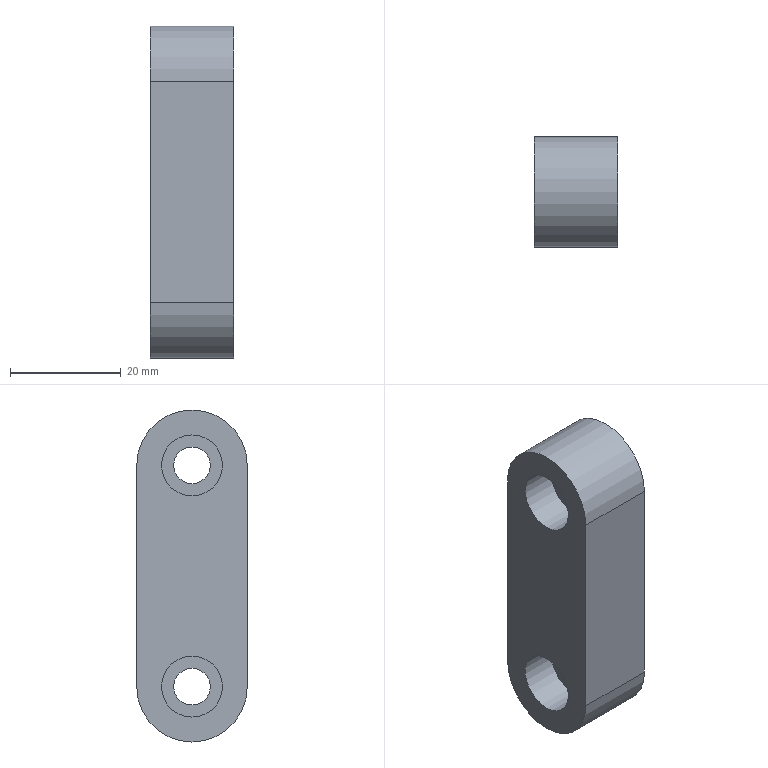Component | NX | SLIDER | 1 solid | 12 faces | box 15 x 20 x 60 mm | volume 14859 mm3 | plane 6 | cylinder 6 | commonest cylinder face diameters 6.6 x2 11 x2 20 x2
STEP:
#1=CARTESIAN_POINT('',(0.,0.,0.));
#2=DIRECTION('',(0.,0.,1.));
#3=DIRECTION('',(1.,0.,0.));
#4=AXIS2_PLACEMENT_3D('',#1,#2,#3);
#5=CARTESIAN_POINT('',(495.625,-9.909,-94.557));
#6=VERTEX_POINT('',#5);
#7=CARTESIAN_POINT('',(495.625,-9.909,-134.557));
#8=VERTEX_POINT('',#7);
#9=CARTESIAN_POINT('',(495.625,-9.909,-84.557));
#10=DIRECTION('',(0.,0.,-1.));
#11=VECTOR('',#10,1.);
#12=LINE('',#9,#11);
#13=CARTESIAN_POINT('',(510.625,-9.909,-84.557));
#14=DIRECTION('',(0.,1.,0.));
#15=DIRECTION('',(0.,0.,1.));
#16=AXIS2_PLACEMENT_3D('',#13,#14,#15);
#17=PLANE('',#16);
#18=CARTESIAN_POINT('',(0.,-15.));
#19=DIRECTION('',(-1.,0.));
#20=VECTOR('',#19,1.);
#21=LINE('',#18,#20);
#22=(GEOMETRIC_REPRESENTATION_CONTEXT(2)PARAMETRIC_REPRESENTATION_CONTEXT()REPRESENTATION_CONTEXT('',''));
#23=DEFINITIONAL_REPRESENTATION('',(#21),#22);
#24=PCURVE('',#17,#23);
#25=CARTESIAN_POINT('',(495.625,0.09065,-114.557));
#26=DIRECTION('',(1.,0.,0.));
#27=DIRECTION('',(0.,0.,-1.));
#28=AXIS2_PLACEMENT_3D('',#25,#26,#27);
#29=PLANE('',#28);
#30=CARTESIAN_POINT('',(-30.,-10.));
#31=DIRECTION('',(1.,0.));
#32=VECTOR('',#31,1.);
#33=LINE('',#30,#32);
#34=(GEOMETRIC_REPRESENTATION_CONTEXT(2)PARAMETRIC_REPRESENTATION_CONTEXT()REPRESENTATION_CONTEXT('',''));
#35=DEFINITIONAL_REPRESENTATION('',(#33),#34);
#36=PCURVE('',#29,#35);
#37=SURFACE_CURVE('',#12,(#24,#36),.PCURVE_S1.);
#38=EDGE_CURVE('',#6,#8,#37,.T.);
#39=ORIENTED_EDGE('',*,*,#38,.T.);
#40=CARTESIAN_POINT('',(510.625,-9.909,-134.557));
#41=VERTEX_POINT('',#40);
#42=CARTESIAN_POINT('',(510.625,-9.909,-134.557));
#43=DIRECTION('',(1.,0.,0.));
#44=VECTOR('',#43,1.);
#45=LINE('',#42,#44);
#46=CARTESIAN_POINT('',(-50.,0.));
#47=DIRECTION('',(0.,1.));
#48=VECTOR('',#47,1.);
#49=LINE('',#46,#48);
#50=(GEOMETRIC_REPRESENTATION_CONTEXT(2)PARAMETRIC_REPRESENTATION_CONTEXT()REPRESENTATION_CONTEXT('',''));
#51=DEFINITIONAL_REPRESENTATION('',(#49),#50);
#52=PCURVE('',#17,#51);
#53=CARTESIAN_POINT('',(510.625,0.09065,-134.557));
#54=DIRECTION('',(-1.,0.,0.));
#55=DIRECTION('',(0.,0.,1.));
#56=AXIS2_PLACEMENT_3D('',#53,#54,#55);
#57=CYLINDRICAL_SURFACE('',#56,10.);
#58=CARTESIAN_POINT('',(4.712,0.));
#59=DIRECTION('',(0.,-1.));
#60=VECTOR('',#59,1.);
#61=LINE('',#58,#60);
#62=(GEOMETRIC_REPRESENTATION_CONTEXT(2)PARAMETRIC_REPRESENTATION_CONTEXT()REPRESENTATION_CONTEXT('',''));
#63=DEFINITIONAL_REPRESENTATION('',(#61),#62);
#64=PCURVE('',#57,#63);
#65=SURFACE_CURVE('',#45,(#52,#64),.PCURVE_S1.);
#66=EDGE_CURVE('',#8,#41,#65,.T.);
#67=ORIENTED_EDGE('',*,*,#66,.T.);
#68=CARTESIAN_POINT('',(510.625,-9.909,-94.557));
#69=VERTEX_POINT('',#68);
#70=CARTESIAN_POINT('',(510.625,-9.909,-84.557));
#71=DIRECTION('',(0.,0.,-1.));
#72=VECTOR('',#71,1.);
#73=LINE('',#70,#72);
#74=CARTESIAN_POINT('',(0.,0.));
#75=DIRECTION('',(-1.,0.));
#76=VECTOR('',#75,1.);
#77=LINE('',#74,#76);
#78=(GEOMETRIC_REPRESENTATION_CONTEXT(2)PARAMETRIC_REPRESENTATION_CONTEXT()REPRESENTATION_CONTEXT('',''));
#79=DEFINITIONAL_REPRESENTATION('',(#77),#78);
#80=PCURVE('',#17,#79);
#81=CARTESIAN_POINT('',(510.625,0.09065,-114.557));
#82=DIRECTION('',(1.,0.,0.));
#83=DIRECTION('',(0.,0.,-1.));
#84=AXIS2_PLACEMENT_3D('',#81,#82,#83);
#85=PLANE('',#84);
#86=CARTESIAN_POINT('',(-30.,-10.));
#87=DIRECTION('',(1.,0.));
#88=VECTOR('',#87,1.);
#89=LINE('',#86,#88);
#90=(GEOMETRIC_REPRESENTATION_CONTEXT(2)PARAMETRIC_REPRESENTATION_CONTEXT()REPRESENTATION_CONTEXT('',''));
#91=DEFINITIONAL_REPRESENTATION('',(#89),#90);
#92=PCURVE('',#85,#91);
#93=SURFACE_CURVE('',#73,(#80,#92),.PCURVE_S1.);
#94=EDGE_CURVE('',#69,#41,#93,.T.);
#95=ORIENTED_EDGE('',*,*,#94,.F.);
#96=CARTESIAN_POINT('',(510.625,-9.909,-94.557));
#97=DIRECTION('',(-1.,0.,0.));
#98=VECTOR('',#97,1.);
#99=LINE('',#96,#98);
#100=CARTESIAN_POINT('',(-10.,0.));
#101=DIRECTION('',(0.,-1.));
#102=VECTOR('',#101,1.);
#103=LINE('',#100,#102);
#104=(GEOMETRIC_REPRESENTATION_CONTEXT(2)PARAMETRIC_REPRESENTATION_CONTEXT()REPRESENTATION_CONTEXT('',''));
#105=DEFINITIONAL_REPRESENTATION('',(#103),#104);
#106=PCURVE('',#17,#105);
#107=CARTESIAN_POINT('',(510.625,0.09065,-94.557));
#108=DIRECTION('',(-1.,0.,0.));
#109=DIRECTION('',(0.,0.,1.));
#110=AXIS2_PLACEMENT_3D('',#107,#108,#109);
#111=CYLINDRICAL_SURFACE('',#110,10.);
#112=CARTESIAN_POINT('',(4.712,0.));
#113=DIRECTION('',(0.,1.));
#114=VECTOR('',#113,1.);
#115=LINE('',#112,#114);
#116=(GEOMETRIC_REPRESENTATION_CONTEXT(2)PARAMETRIC_REPRESENTATION_CONTEXT()REPRESENTATION_CONTEXT('',''));
#117=DEFINITIONAL_REPRESENTATION('',(#115),#116);
#118=PCURVE('',#111,#117);
#119=SURFACE_CURVE('',#99,(#106,#118),.PCURVE_S1.);
#120=EDGE_CURVE('',#69,#6,#119,.T.);
#121=ORIENTED_EDGE('',*,*,#120,.T.);
#122=EDGE_LOOP('',(#39,#67,#95,#121));
#123=FACE_BOUND('',#122,.T.);
#124=ADVANCED_FACE('',(#123),#17,.F.);
#125=CARTESIAN_POINT('',(510.625,10.091,-134.557));
#126=VERTEX_POINT('',#125);
#127=CARTESIAN_POINT('',(510.625,10.091,-94.557));
#128=VERTEX_POINT('',#127);
#129=CARTESIAN_POINT('',(510.625,10.091,-144.557));
#130=DIRECTION('',(0.,0.,1.));
#131=VECTOR('',#130,1.);
#132=LINE('',#129,#131);
#133=CARTESIAN_POINT('',(510.625,10.091,-144.557));
#134=DIRECTION('',(0.,-1.,0.));
#135=DIRECTION('',(0.,0.,-1.));
#136=AXIS2_PLACEMENT_3D('',#133,#134,#135);
#137=PLANE('',#136);
#138=CARTESIAN_POINT('',(0.,0.));
#139=DIRECTION('',(-1.,0.));
#140=VECTOR('',#139,1.);
#141=LINE('',#138,#140);
#142=(GEOMETRIC_REPRESENTATION_CONTEXT(2)PARAMETRIC_REPRESENTATION_CONTEXT()REPRESENTATION_CONTEXT('',''));
#143=DEFINITIONAL_REPRESENTATION('',(#141),#142);
#144=PCURVE('',#137,#143);
#145=CARTESIAN_POINT('',(30.,10.));
#146=DIRECTION('',(-1.,0.));
#147=VECTOR('',#146,1.);
#148=LINE('',#145,#147);
#149=(GEOMETRIC_REPRESENTATION_CONTEXT(2)PARAMETRIC_REPRESENTATION_CONTEXT()REPRESENTATION_CONTEXT('',''));
#150=DEFINITIONAL_REPRESENTATION('',(#148),#149);
#151=PCURVE('',#85,#150);
#152=SURFACE_CURVE('',#132,(#144,#151),.PCURVE_S1.);
#153=EDGE_CURVE('',#126,#128,#152,.T.);
#154=ORIENTED_EDGE('',*,*,#153,.F.);
#155=CARTESIAN_POINT('',(495.625,10.091,-134.557));
#156=VERTEX_POINT('',#155);
#157=CARTESIAN_POINT('',(510.625,10.091,-134.557));
#158=DIRECTION('',(-1.,0.,0.));
#159=VECTOR('',#158,1.);
#160=LINE('',#157,#159);
#161=CARTESIAN_POINT('',(-10.,0.));
#162=DIRECTION('',(0.,-1.));
#163=VECTOR('',#162,1.);
#164=LINE('',#161,#163);
#165=(GEOMETRIC_REPRESENTATION_CONTEXT(2)PARAMETRIC_REPRESENTATION_CONTEXT()REPRESENTATION_CONTEXT('',''));
#166=DEFINITIONAL_REPRESENTATION('',(#164),#165);
#167=PCURVE('',#137,#166);
#168=CARTESIAN_POINT('',(1.571,0.));
#169=DIRECTION('',(0.,1.));
#170=VECTOR('',#169,1.);
#171=LINE('',#168,#170);
#172=(GEOMETRIC_REPRESENTATION_CONTEXT(2)PARAMETRIC_REPRESENTATION_CONTEXT()REPRESENTATION_CONTEXT('',''));
#173=DEFINITIONAL_REPRESENTATION('',(#171),#172);
#174=PCURVE('',#57,#173);
#175=SURFACE_CURVE('',#160,(#167,#174),.PCURVE_S1.);
#176=EDGE_CURVE('',#126,#156,#175,.T.);
#177=ORIENTED_EDGE('',*,*,#176,.T.);
#178=CARTESIAN_POINT('',(495.625,10.091,-94.557));
#179=VERTEX_POINT('',#178);
#180=CARTESIAN_POINT('',(495.625,10.091,-144.557));
#181=DIRECTION('',(0.,0.,1.));
#182=VECTOR('',#181,1.);
#183=LINE('',#180,#182);
#184=CARTESIAN_POINT('',(0.,-15.));
#185=DIRECTION('',(-1.,0.));
#186=VECTOR('',#185,1.);
#187=LINE('',#184,#186);
#188=(GEOMETRIC_REPRESENTATION_CONTEXT(2)PARAMETRIC_REPRESENTATION_CONTEXT()REPRESENTATION_CONTEXT('',''));
#189=DEFINITIONAL_REPRESENTATION('',(#187),#188);
#190=PCURVE('',#137,#189);
#191=CARTESIAN_POINT('',(30.,10.));
#192=DIRECTION('',(-1.,0.));
#193=VECTOR('',#192,1.);
#194=LINE('',#191,#193);
#195=(GEOMETRIC_REPRESENTATION_CONTEXT(2)PARAMETRIC_REPRESENTATION_CONTEXT()REPRESENTATION_CONTEXT('',''));
#196=DEFINITIONAL_REPRESENTATION('',(#194),#195);
#197=PCURVE('',#29,#196);
#198=SURFACE_CURVE('',#183,(#190,#197),.PCURVE_S1.);
#199=EDGE_CURVE('',#156,#179,#198,.T.);
#200=ORIENTED_EDGE('',*,*,#199,.T.);
#201=CARTESIAN_POINT('',(510.625,10.091,-94.557));
#202=DIRECTION('',(1.,0.,0.));
#203=VECTOR('',#202,1.);
#204=LINE('',#201,#203);
#205=CARTESIAN_POINT('',(-50.,0.));
#206=DIRECTION('',(0.,1.));
#207=VECTOR('',#206,1.);
#208=LINE('',#205,#207);
#209=(GEOMETRIC_REPRESENTATION_CONTEXT(2)PARAMETRIC_REPRESENTATION_CONTEXT()REPRESENTATION_CONTEXT('',''));
#210=DEFINITIONAL_REPRESENTATION('',(#208),#209);
#211=PCURVE('',#137,#210);
#212=CARTESIAN_POINT('',(7.854,0.));
#213=DIRECTION('',(0.,-1.));
#214=VECTOR('',#213,1.);
#215=LINE('',#212,#214);
#216=(GEOMETRIC_REPRESENTATION_CONTEXT(2)PARAMETRIC_REPRESENTATION_CONTEXT()REPRESENTATION_CONTEXT('',''));
#217=DEFINITIONAL_REPRESENTATION('',(#215),#216);
#218=PCURVE('',#111,#217);
#219=SURFACE_CURVE('',#204,(#211,#218),.PCURVE_S1.);
#220=EDGE_CURVE('',#179,#128,#219,.T.);
#221=ORIENTED_EDGE('',*,*,#220,.T.);
#222=EDGE_LOOP('',(#154,#177,#200,#221));
#223=FACE_BOUND('',#222,.T.);
#224=ADVANCED_FACE('',(#223),#137,.F.);
#225=CARTESIAN_POINT('',(510.625,0.09065,-97.857));
#226=VERTEX_POINT('',#225);
#227=CARTESIAN_POINT('',(510.625,0.09065,-94.557));
#228=DIRECTION('',(1.,0.,0.));
#229=DIRECTION('',(0.,0.,-1.));
#230=AXIS2_PLACEMENT_3D('',#227,#228,#229);
#231=CIRCLE('',#230,3.3);
#232=CARTESIAN_POINT('',(-20.,0.));
#233=DIRECTION('',(1.,0.));
#234=AXIS2_PLACEMENT_2D('',#232,#233);
#235=CIRCLE('',#234,3.3);
#236=(GEOMETRIC_REPRESENTATION_CONTEXT(2)PARAMETRIC_REPRESENTATION_CONTEXT()REPRESENTATION_CONTEXT('',''));
#237=DEFINITIONAL_REPRESENTATION('',(#235),#236);
#238=PCURVE('',#85,#237);
#239=CARTESIAN_POINT('',(532.757,0.09065,-94.557));
#240=DIRECTION('',(1.,0.,0.));
#241=DIRECTION('',(0.,0.,-1.));
#242=AXIS2_PLACEMENT_3D('',#239,#240,#241);
#243=CYLINDRICAL_SURFACE('',#242,3.3);
#244=CARTESIAN_POINT('',(0.,-22.132));
#245=DIRECTION('',(1.,0.));
#246=VECTOR('',#245,1.);
#247=LINE('',#244,#246);
#248=(GEOMETRIC_REPRESENTATION_CONTEXT(2)PARAMETRIC_REPRESENTATION_CONTEXT()REPRESENTATION_CONTEXT('',''));
#249=DEFINITIONAL_REPRESENTATION('',(#247),#248);
#250=PCURVE('',#243,#249);
#251=SURFACE_CURVE('',#231,(#238,#250),.PCURVE_S1.);
#252=EDGE_CURVE('',#226,#226,#251,.T.);
#253=ORIENTED_EDGE('',*,*,#252,.F.);
#254=EDGE_LOOP('',(#253));
#255=FACE_BOUND('',#254,.T.);
#256=CARTESIAN_POINT('',(510.625,0.09065,-137.857));
#257=VERTEX_POINT('',#256);
#258=CARTESIAN_POINT('',(510.625,0.09065,-134.557));
#259=DIRECTION('',(1.,0.,0.));
#260=DIRECTION('',(0.,0.,-1.));
#261=AXIS2_PLACEMENT_3D('',#258,#259,#260);
#262=CIRCLE('',#261,3.3);
#263=CARTESIAN_POINT('',(20.,0.));
#264=DIRECTION('',(1.,0.));
#265=AXIS2_PLACEMENT_2D('',#263,#264);
#266=CIRCLE('',#265,3.3);
#267=(GEOMETRIC_REPRESENTATION_CONTEXT(2)PARAMETRIC_REPRESENTATION_CONTEXT()REPRESENTATION_CONTEXT('',''));
#268=DEFINITIONAL_REPRESENTATION('',(#266),#267);
#269=PCURVE('',#85,#268);
#270=CARTESIAN_POINT('',(532.757,0.09065,-134.557));
#271=DIRECTION('',(1.,0.,0.));
#272=DIRECTION('',(0.,0.,-1.));
#273=AXIS2_PLACEMENT_3D('',#270,#271,#272);
#274=CYLINDRICAL_SURFACE('',#273,3.3);
#275=CARTESIAN_POINT('',(0.,-22.132));
#276=DIRECTION('',(1.,0.));
#277=VECTOR('',#276,1.);
#278=LINE('',#275,#277);
#279=(GEOMETRIC_REPRESENTATION_CONTEXT(2)PARAMETRIC_REPRESENTATION_CONTEXT()REPRESENTATION_CONTEXT('',''));
#280=DEFINITIONAL_REPRESENTATION('',(#278),#279);
#281=PCURVE('',#274,#280);
#282=SURFACE_CURVE('',#262,(#269,#281),.PCURVE_S1.);
#283=EDGE_CURVE('',#257,#257,#282,.T.);
#284=ORIENTED_EDGE('',*,*,#283,.F.);
#285=EDGE_LOOP('',(#284));
#286=FACE_BOUND('',#285,.T.);
#287=CARTESIAN_POINT('',(510.625,0.09065,-134.557));
#288=DIRECTION('',(1.,0.,0.));
#289=DIRECTION('',(0.,0.,-1.));
#290=AXIS2_PLACEMENT_3D('',#287,#288,#289);
#291=CIRCLE('',#290,10.);
#292=CARTESIAN_POINT('',(20.,-0.));
#293=DIRECTION('',(1.,0.));
#294=AXIS2_PLACEMENT_2D('',#292,#293);
#295=CIRCLE('',#294,10.);
#296=(GEOMETRIC_REPRESENTATION_CONTEXT(2)PARAMETRIC_REPRESENTATION_CONTEXT()REPRESENTATION_CONTEXT('',''));
#297=DEFINITIONAL_REPRESENTATION('',(#295),#296);
#298=PCURVE('',#85,#297);
#299=CARTESIAN_POINT('',(9.425,0.));
#300=DIRECTION('',(-1.,0.));
#301=VECTOR('',#300,1.);
#302=LINE('',#299,#301);
#303=(GEOMETRIC_REPRESENTATION_CONTEXT(2)PARAMETRIC_REPRESENTATION_CONTEXT()REPRESENTATION_CONTEXT('',''));
#304=DEFINITIONAL_REPRESENTATION('',(#302),#303);
#305=PCURVE('',#57,#304);
#306=SURFACE_CURVE('',#291,(#298,#305),.PCURVE_S1.);
#307=EDGE_CURVE('',#41,#126,#306,.T.);
#308=ORIENTED_EDGE('',*,*,#307,.T.);
#309=ORIENTED_EDGE('',*,*,#153,.T.);
#310=CARTESIAN_POINT('',(510.625,0.09065,-94.557));
#311=DIRECTION('',(1.,0.,0.));
#312=DIRECTION('',(0.,0.,-1.));
#313=AXIS2_PLACEMENT_3D('',#310,#311,#312);
#314=CIRCLE('',#313,10.);
#315=CARTESIAN_POINT('',(-20.,0.));
#316=DIRECTION('',(1.,0.));
#317=AXIS2_PLACEMENT_2D('',#315,#316);
#318=CIRCLE('',#317,10.);
#319=(GEOMETRIC_REPRESENTATION_CONTEXT(2)PARAMETRIC_REPRESENTATION_CONTEXT()REPRESENTATION_CONTEXT('',''));
#320=DEFINITIONAL_REPRESENTATION('',(#318),#319);
#321=PCURVE('',#85,#320);
#322=CARTESIAN_POINT('',(9.425,0.));
#323=DIRECTION('',(-1.,0.));
#324=VECTOR('',#323,1.);
#325=LINE('',#322,#324);
#326=(GEOMETRIC_REPRESENTATION_CONTEXT(2)PARAMETRIC_REPRESENTATION_CONTEXT()REPRESENTATION_CONTEXT('',''));
#327=DEFINITIONAL_REPRESENTATION('',(#325),#326);
#328=PCURVE('',#111,#327);
#329=SURFACE_CURVE('',#314,(#321,#328),.PCURVE_S1.);
#330=EDGE_CURVE('',#128,#69,#329,.T.);
#331=ORIENTED_EDGE('',*,*,#330,.T.);
#332=ORIENTED_EDGE('',*,*,#94,.T.);
#333=EDGE_LOOP('',(#308,#309,#331,#332));
#334=FACE_BOUND('',#333,.T.);
#335=ADVANCED_FACE('',(#255,#286,#334),#85,.T.);
#336=CARTESIAN_POINT('',(495.625,0.09065,-100.057));
#337=VERTEX_POINT('',#336);
#338=CARTESIAN_POINT('',(495.625,0.09065,-94.557));
#339=DIRECTION('',(1.,0.,0.));
#340=DIRECTION('',(0.,0.,-1.));
#341=AXIS2_PLACEMENT_3D('',#338,#339,#340);
#342=CIRCLE('',#341,5.5);
#343=CARTESIAN_POINT('',(-20.,0.));
#344=DIRECTION('',(1.,0.));
#345=AXIS2_PLACEMENT_2D('',#343,#344);
#346=CIRCLE('',#345,5.5);
#347=(GEOMETRIC_REPRESENTATION_CONTEXT(2)PARAMETRIC_REPRESENTATION_CONTEXT()REPRESENTATION_CONTEXT('',''));
#348=DEFINITIONAL_REPRESENTATION('',(#346),#347);
#349=PCURVE('',#29,#348);
#350=CARTESIAN_POINT('',(495.625,0.09065,-94.557));
#351=DIRECTION('',(1.,0.,0.));
#352=DIRECTION('',(0.,0.,-1.));
#353=AXIS2_PLACEMENT_3D('',#350,#351,#352);
#354=CYLINDRICAL_SURFACE('',#353,5.5);
#355=CARTESIAN_POINT('',(0.,0.));
#356=DIRECTION('',(1.,0.));
#357=VECTOR('',#356,1.);
#358=LINE('',#355,#357);
#359=(GEOMETRIC_REPRESENTATION_CONTEXT(2)PARAMETRIC_REPRESENTATION_CONTEXT()REPRESENTATION_CONTEXT('',''));
#360=DEFINITIONAL_REPRESENTATION('',(#358),#359);
#361=PCURVE('',#354,#360);
#362=SURFACE_CURVE('',#342,(#349,#361),.PCURVE_S1.);
#363=EDGE_CURVE('',#337,#337,#362,.T.);
#364=ORIENTED_EDGE('',*,*,#363,.T.);
#365=EDGE_LOOP('',(#364));
#366=FACE_BOUND('',#365,.T.);
#367=CARTESIAN_POINT('',(495.625,0.09065,-140.057));
#368=VERTEX_POINT('',#367);
#369=CARTESIAN_POINT('',(495.625,0.09065,-134.557));
#370=DIRECTION('',(1.,0.,0.));
#371=DIRECTION('',(0.,0.,-1.));
#372=AXIS2_PLACEMENT_3D('',#369,#370,#371);
#373=CIRCLE('',#372,5.5);
#374=CARTESIAN_POINT('',(20.,0.));
#375=DIRECTION('',(1.,0.));
#376=AXIS2_PLACEMENT_2D('',#374,#375);
#377=CIRCLE('',#376,5.5);
#378=(GEOMETRIC_REPRESENTATION_CONTEXT(2)PARAMETRIC_REPRESENTATION_CONTEXT()REPRESENTATION_CONTEXT('',''));
#379=DEFINITIONAL_REPRESENTATION('',(#377),#378);
#380=PCURVE('',#29,#379);
#381=CARTESIAN_POINT('',(495.625,0.09065,-134.557));
#382=DIRECTION('',(1.,0.,0.));
#383=DIRECTION('',(0.,0.,-1.));
#384=AXIS2_PLACEMENT_3D('',#381,#382,#383);
#385=CYLINDRICAL_SURFACE('',#384,5.5);
#386=CARTESIAN_POINT('',(0.,0.));
#387=DIRECTION('',(1.,0.));
#388=VECTOR('',#387,1.);
#389=LINE('',#386,#388);
#390=(GEOMETRIC_REPRESENTATION_CONTEXT(2)PARAMETRIC_REPRESENTATION_CONTEXT()REPRESENTATION_CONTEXT('',''));
#391=DEFINITIONAL_REPRESENTATION('',(#389),#390);
#392=PCURVE('',#385,#391);
#393=SURFACE_CURVE('',#373,(#380,#392),.PCURVE_S1.);
#394=EDGE_CURVE('',#368,#368,#393,.T.);
#395=ORIENTED_EDGE('',*,*,#394,.T.);
#396=EDGE_LOOP('',(#395));
#397=FACE_BOUND('',#396,.T.);
#398=ORIENTED_EDGE('',*,*,#199,.F.);
#399=CARTESIAN_POINT('',(495.625,0.09065,-134.557));
#400=DIRECTION('',(-1.,0.,0.));
#401=DIRECTION('',(0.,0.,-1.));
#402=AXIS2_PLACEMENT_3D('',#399,#400,#401);
#403=CIRCLE('',#402,10.);
#404=CARTESIAN_POINT('',(30.,-0.));
#405=CARTESIAN_POINT('',(30.,-17.321));
#406=CARTESIAN_POINT('',(15.,-8.66));
#407=CARTESIAN_POINT('',(-0.,-0.));
#408=CARTESIAN_POINT('',(15.,8.66));
#409=CARTESIAN_POINT('',(30.,17.321));
#410=CARTESIAN_POINT('',(30.,-0.));
#411=(BOUNDED_CURVE()B_SPLINE_CURVE(2,(#404,#405,#406,#407,#408,#409,#410),.UNSPECIFIED.,.T.,.F.)B_SPLINE_CURVE_WITH_KNOTS((1,2,2,2,2,1),(-2.094,0.,2.094,4.189,6.283,8.378),.UNSPECIFIED.)CURVE()GEOMETRIC_REPRESENTATION_ITEM()RATIONAL_B_SPLINE_CURVE((1.,0.5,1.,0.5,1.,0.5,1.))REPRESENTATION_ITEM(''));
#412=(GEOMETRIC_REPRESENTATION_CONTEXT(2)PARAMETRIC_REPRESENTATION_CONTEXT()REPRESENTATION_CONTEXT('',''));
#413=DEFINITIONAL_REPRESENTATION('',(#411),#412);
#414=PCURVE('',#29,#413);
#415=CARTESIAN_POINT('',(-3.142,15.));
#416=DIRECTION('',(1.,0.));
#417=VECTOR('',#416,1.);
#418=LINE('',#415,#417);
#419=(GEOMETRIC_REPRESENTATION_CONTEXT(2)PARAMETRIC_REPRESENTATION_CONTEXT()REPRESENTATION_CONTEXT('',''));
#420=DEFINITIONAL_REPRESENTATION('',(#418),#419);
#421=PCURVE('',#57,#420);
#422=SURFACE_CURVE('',#403,(#414,#421),.PCURVE_S1.);
#423=EDGE_CURVE('',#156,#8,#422,.T.);
#424=ORIENTED_EDGE('',*,*,#423,.T.);
#425=ORIENTED_EDGE('',*,*,#38,.F.);
#426=CARTESIAN_POINT('',(495.625,0.09065,-94.557));
#427=DIRECTION('',(-1.,0.,0.));
#428=DIRECTION('',(0.,0.,-1.));
#429=AXIS2_PLACEMENT_3D('',#426,#427,#428);
#430=CIRCLE('',#429,10.);
#431=CARTESIAN_POINT('',(-10.,0.));
#432=CARTESIAN_POINT('',(-10.,-17.321));
#433=CARTESIAN_POINT('',(-25.,-8.66));
#434=CARTESIAN_POINT('',(-40.,0.));
#435=CARTESIAN_POINT('',(-25.,8.66));
#436=CARTESIAN_POINT('',(-10.,17.321));
#437=CARTESIAN_POINT('',(-10.,0.));
#438=(BOUNDED_CURVE()B_SPLINE_CURVE(2,(#431,#432,#433,#434,#435,#436,#437),.UNSPECIFIED.,.T.,.F.)B_SPLINE_CURVE_WITH_KNOTS((1,2,2,2,2,1),(-2.094,0.,2.094,4.189,6.283,8.378),.UNSPECIFIED.)CURVE()GEOMETRIC_REPRESENTATION_ITEM()RATIONAL_B_SPLINE_CURVE((1.,0.5,1.,0.5,1.,0.5,1.))REPRESENTATION_ITEM(''));
#439=(GEOMETRIC_REPRESENTATION_CONTEXT(2)PARAMETRIC_REPRESENTATION_CONTEXT()REPRESENTATION_CONTEXT('',''));
#440=DEFINITIONAL_REPRESENTATION('',(#438),#439);
#441=PCURVE('',#29,#440);
#442=CARTESIAN_POINT('',(3.142,15.));
#443=DIRECTION('',(1.,0.));
#444=VECTOR('',#443,1.);
#445=LINE('',#442,#444);
#446=(GEOMETRIC_REPRESENTATION_CONTEXT(2)PARAMETRIC_REPRESENTATION_CONTEXT()REPRESENTATION_CONTEXT('',''));
#447=DEFINITIONAL_REPRESENTATION('',(#445),#446);
#448=PCURVE('',#111,#447);
#449=SURFACE_CURVE('',#430,(#441,#448),.PCURVE_S1.);
#450=EDGE_CURVE('',#6,#179,#449,.T.);
#451=ORIENTED_EDGE('',*,*,#450,.T.);
#452=EDGE_LOOP('',(#398,#424,#425,#451));
#453=FACE_BOUND('',#452,.T.);
#454=ADVANCED_FACE('',(#366,#397,#453),#29,.F.);
#455=ORIENTED_EDGE('',*,*,#283,.F.);
#456=CARTESIAN_POINT('',(502.425,0.09065,-137.857));
#457=VERTEX_POINT('',#456);
#458=CARTESIAN_POINT('',(502.425,0.09065,-137.857));
#459=CARTESIAN_POINT('',(510.625,0.09065,-137.857));
#460=B_SPLINE_CURVE_WITH_KNOTS('',1,(#458,#459),.UNSPECIFIED.,.F.,.F.,(2,2),(-30.332,-22.132),.PIECEWISE_BEZIER_KNOTS.);
#461=CARTESIAN_POINT('',(0.,0.));
#462=DIRECTION('',(0.,1.));
#463=VECTOR('',#462,1.);
#464=LINE('',#461,#463);
#465=(GEOMETRIC_REPRESENTATION_CONTEXT(2)PARAMETRIC_REPRESENTATION_CONTEXT()REPRESENTATION_CONTEXT('',''));
#466=DEFINITIONAL_REPRESENTATION('',(#464),#465);
#467=PCURVE('',#274,#466);
#468=CARTESIAN_POINT('',(6.283,0.));
#469=DIRECTION('',(0.,1.));
#470=VECTOR('',#469,1.);
#471=LINE('',#468,#470);
#472=(GEOMETRIC_REPRESENTATION_CONTEXT(2)PARAMETRIC_REPRESENTATION_CONTEXT()REPRESENTATION_CONTEXT('',''));
#473=DEFINITIONAL_REPRESENTATION('',(#471),#472);
#474=PCURVE('',#274,#473);
#475=SEAM_CURVE('',#460,(#467,#474),.PCURVE_S1.);
#476=EDGE_CURVE('',#457,#257,#475,.T.);
#477=ORIENTED_EDGE('',*,*,#476,.F.);
#478=CARTESIAN_POINT('',(502.425,0.09065,-134.557));
#479=DIRECTION('',(-1.,0.,0.));
#480=DIRECTION('',(0.,0.,-1.));
#481=AXIS2_PLACEMENT_3D('',#478,#479,#480);
#482=CIRCLE('',#481,3.3);
#483=CARTESIAN_POINT('',(6.283,-30.332));
#484=DIRECTION('',(-1.,0.));
#485=VECTOR('',#484,1.);
#486=LINE('',#483,#485);
#487=(GEOMETRIC_REPRESENTATION_CONTEXT(2)PARAMETRIC_REPRESENTATION_CONTEXT()REPRESENTATION_CONTEXT('',''));
#488=DEFINITIONAL_REPRESENTATION('',(#486),#487);
#489=PCURVE('',#274,#488);
#490=CARTESIAN_POINT('',(502.425,0.09065,-134.557));
#491=DIRECTION('',(1.,0.,0.));
#492=DIRECTION('',(0.,0.,-1.));
#493=AXIS2_PLACEMENT_3D('',#490,#491,#492);
#494=PLANE('',#493);
#495=CARTESIAN_POINT('',(3.3,0.));
#496=CARTESIAN_POINT('',(3.3,-5.716));
#497=CARTESIAN_POINT('',(-1.65,-2.858));
#498=CARTESIAN_POINT('',(-6.6,-0.));
#499=CARTESIAN_POINT('',(-1.65,2.858));
#500=CARTESIAN_POINT('',(3.3,5.716));
#501=CARTESIAN_POINT('',(3.3,0.));
#502=(BOUNDED_CURVE()B_SPLINE_CURVE(2,(#495,#496,#497,#498,#499,#500,#501),.UNSPECIFIED.,.T.,.F.)B_SPLINE_CURVE_WITH_KNOTS((1,2,2,2,2,1),(-2.094,0.,2.094,4.189,6.283,8.378),.UNSPECIFIED.)CURVE()GEOMETRIC_REPRESENTATION_ITEM()RATIONAL_B_SPLINE_CURVE((1.,0.5,1.,0.5,1.,0.5,1.))REPRESENTATION_ITEM(''));
#503=(GEOMETRIC_REPRESENTATION_CONTEXT(2)PARAMETRIC_REPRESENTATION_CONTEXT()REPRESENTATION_CONTEXT('',''));
#504=DEFINITIONAL_REPRESENTATION('',(#502),#503);
#505=PCURVE('',#494,#504);
#506=SURFACE_CURVE('',#482,(#489,#505),.PCURVE_S1.);
#507=EDGE_CURVE('',#457,#457,#506,.T.);
#508=ORIENTED_EDGE('',*,*,#507,.F.);
#509=ORIENTED_EDGE('',*,*,#476,.T.);
#510=EDGE_LOOP('',(#455,#477,#508,#509));
#511=FACE_BOUND('',#510,.F.);
#512=ADVANCED_FACE('',(#511),#274,.F.);
#513=ORIENTED_EDGE('',*,*,#507,.F.);
#514=EDGE_LOOP('',(#513));
#515=FACE_BOUND('',#514,.T.);
#516=CARTESIAN_POINT('',(502.425,0.09065,-140.057));
#517=VERTEX_POINT('',#516);
#518=CARTESIAN_POINT('',(502.425,0.09065,-134.557));
#519=DIRECTION('',(-1.,0.,0.));
#520=DIRECTION('',(0.,0.,-1.));
#521=AXIS2_PLACEMENT_3D('',#518,#519,#520);
#522=CIRCLE('',#521,5.5);
#523=CARTESIAN_POINT('',(5.5,0.));
#524=CARTESIAN_POINT('',(5.5,-9.526));
#525=CARTESIAN_POINT('',(-2.75,-4.763));
#526=CARTESIAN_POINT('',(-11.,-0.));
#527=CARTESIAN_POINT('',(-2.75,4.763));
#528=CARTESIAN_POINT('',(5.5,9.526));
#529=CARTESIAN_POINT('',(5.5,0.));
#530=(BOUNDED_CURVE()B_SPLINE_CURVE(2,(#523,#524,#525,#526,#527,#528,#529),.UNSPECIFIED.,.T.,.F.)B_SPLINE_CURVE_WITH_KNOTS((1,2,2,2,2,1),(-2.094,0.,2.094,4.189,6.283,8.378),.UNSPECIFIED.)CURVE()GEOMETRIC_REPRESENTATION_ITEM()RATIONAL_B_SPLINE_CURVE((1.,0.5,1.,0.5,1.,0.5,1.))REPRESENTATION_ITEM(''));
#531=(GEOMETRIC_REPRESENTATION_CONTEXT(2)PARAMETRIC_REPRESENTATION_CONTEXT()REPRESENTATION_CONTEXT('',''));
#532=DEFINITIONAL_REPRESENTATION('',(#530),#531);
#533=PCURVE('',#494,#532);
#534=CARTESIAN_POINT('',(6.283,6.8));
#535=DIRECTION('',(-1.,0.));
#536=VECTOR('',#535,1.);
#537=LINE('',#534,#536);
#538=(GEOMETRIC_REPRESENTATION_CONTEXT(2)PARAMETRIC_REPRESENTATION_CONTEXT()REPRESENTATION_CONTEXT('',''));
#539=DEFINITIONAL_REPRESENTATION('',(#537),#538);
#540=PCURVE('',#385,#539);
#541=SURFACE_CURVE('',#522,(#533,#540),.PCURVE_S1.);
#542=EDGE_CURVE('',#517,#517,#541,.T.);
#543=ORIENTED_EDGE('',*,*,#542,.T.);
#544=EDGE_LOOP('',(#543));
#545=FACE_BOUND('',#544,.T.);
#546=ADVANCED_FACE('',(#515,#545),#494,.F.);
#547=ORIENTED_EDGE('',*,*,#542,.T.);
#548=CARTESIAN_POINT('',(495.625,0.09065,-140.057));
#549=CARTESIAN_POINT('',(502.425,0.09065,-140.057));
#550=B_SPLINE_CURVE_WITH_KNOTS('',1,(#548,#549),.UNSPECIFIED.,.F.,.F.,(2,2),(0.,6.8),.PIECEWISE_BEZIER_KNOTS.);
#551=CARTESIAN_POINT('',(0.,0.));
#552=DIRECTION('',(0.,1.));
#553=VECTOR('',#552,1.);
#554=LINE('',#551,#553);
#555=(GEOMETRIC_REPRESENTATION_CONTEXT(2)PARAMETRIC_REPRESENTATION_CONTEXT()REPRESENTATION_CONTEXT('',''));
#556=DEFINITIONAL_REPRESENTATION('',(#554),#555);
#557=PCURVE('',#385,#556);
#558=CARTESIAN_POINT('',(6.283,0.));
#559=DIRECTION('',(0.,1.));
#560=VECTOR('',#559,1.);
#561=LINE('',#558,#560);
#562=(GEOMETRIC_REPRESENTATION_CONTEXT(2)PARAMETRIC_REPRESENTATION_CONTEXT()REPRESENTATION_CONTEXT('',''));
#563=DEFINITIONAL_REPRESENTATION('',(#561),#562);
#564=PCURVE('',#385,#563);
#565=SEAM_CURVE('',#550,(#557,#564),.PCURVE_S1.);
#566=EDGE_CURVE('',#368,#517,#565,.T.);
#567=ORIENTED_EDGE('',*,*,#566,.F.);
#568=ORIENTED_EDGE('',*,*,#394,.T.);
#569=ORIENTED_EDGE('',*,*,#566,.T.);
#570=EDGE_LOOP('',(#547,#567,#568,#569));
#571=FACE_BOUND('',#570,.F.);
#572=ADVANCED_FACE('',(#571),#385,.F.);
#573=ORIENTED_EDGE('',*,*,#252,.F.);
#574=CARTESIAN_POINT('',(502.425,0.09065,-97.857));
#575=VERTEX_POINT('',#574);
#576=CARTESIAN_POINT('',(502.425,0.09065,-97.857));
#577=CARTESIAN_POINT('',(510.625,0.09065,-97.857));
#578=B_SPLINE_CURVE_WITH_KNOTS('',1,(#576,#577),.UNSPECIFIED.,.F.,.F.,(2,2),(-30.332,-22.132),.PIECEWISE_BEZIER_KNOTS.);
#579=CARTESIAN_POINT('',(0.,0.));
#580=DIRECTION('',(0.,1.));
#581=VECTOR('',#580,1.);
#582=LINE('',#579,#581);
#583=(GEOMETRIC_REPRESENTATION_CONTEXT(2)PARAMETRIC_REPRESENTATION_CONTEXT()REPRESENTATION_CONTEXT('',''));
#584=DEFINITIONAL_REPRESENTATION('',(#582),#583);
#585=PCURVE('',#243,#584);
#586=CARTESIAN_POINT('',(6.283,0.));
#587=DIRECTION('',(0.,1.));
#588=VECTOR('',#587,1.);
#589=LINE('',#586,#588);
#590=(GEOMETRIC_REPRESENTATION_CONTEXT(2)PARAMETRIC_REPRESENTATION_CONTEXT()REPRESENTATION_CONTEXT('',''));
#591=DEFINITIONAL_REPRESENTATION('',(#589),#590);
#592=PCURVE('',#243,#591);
#593=SEAM_CURVE('',#578,(#585,#592),.PCURVE_S1.);
#594=EDGE_CURVE('',#575,#226,#593,.T.);
#595=ORIENTED_EDGE('',*,*,#594,.F.);
#596=CARTESIAN_POINT('',(502.425,0.09065,-94.557));
#597=DIRECTION('',(-1.,0.,0.));
#598=DIRECTION('',(0.,0.,-1.));
#599=AXIS2_PLACEMENT_3D('',#596,#597,#598);
#600=CIRCLE('',#599,3.3);
#601=CARTESIAN_POINT('',(6.283,-30.332));
#602=DIRECTION('',(-1.,0.));
#603=VECTOR('',#602,1.);
#604=LINE('',#601,#603);
#605=(GEOMETRIC_REPRESENTATION_CONTEXT(2)PARAMETRIC_REPRESENTATION_CONTEXT()REPRESENTATION_CONTEXT('',''));
#606=DEFINITIONAL_REPRESENTATION('',(#604),#605);
#607=PCURVE('',#243,#606);
#608=CARTESIAN_POINT('',(502.425,0.09065,-94.557));
#609=DIRECTION('',(1.,0.,0.));
#610=DIRECTION('',(0.,0.,-1.));
#611=AXIS2_PLACEMENT_3D('',#608,#609,#610);
#612=PLANE('',#611);
#613=CARTESIAN_POINT('',(3.3,0.));
#614=CARTESIAN_POINT('',(3.3,-5.716));
#615=CARTESIAN_POINT('',(-1.65,-2.858));
#616=CARTESIAN_POINT('',(-6.6,-0.));
#617=CARTESIAN_POINT('',(-1.65,2.858));
#618=CARTESIAN_POINT('',(3.3,5.716));
#619=CARTESIAN_POINT('',(3.3,0.));
#620=(BOUNDED_CURVE()B_SPLINE_CURVE(2,(#613,#614,#615,#616,#617,#618,#619),.UNSPECIFIED.,.T.,.F.)B_SPLINE_CURVE_WITH_KNOTS((1,2,2,2,2,1),(-2.094,0.,2.094,4.189,6.283,8.378),.UNSPECIFIED.)CURVE()GEOMETRIC_REPRESENTATION_ITEM()RATIONAL_B_SPLINE_CURVE((1.,0.5,1.,0.5,1.,0.5,1.))REPRESENTATION_ITEM(''));
#621=(GEOMETRIC_REPRESENTATION_CONTEXT(2)PARAMETRIC_REPRESENTATION_CONTEXT()REPRESENTATION_CONTEXT('',''));
#622=DEFINITIONAL_REPRESENTATION('',(#620),#621);
#623=PCURVE('',#612,#622);
#624=SURFACE_CURVE('',#600,(#607,#623),.PCURVE_S1.);
#625=EDGE_CURVE('',#575,#575,#624,.T.);
#626=ORIENTED_EDGE('',*,*,#625,.F.);
#627=ORIENTED_EDGE('',*,*,#594,.T.);
#628=EDGE_LOOP('',(#573,#595,#626,#627));
#629=FACE_BOUND('',#628,.F.);
#630=ADVANCED_FACE('',(#629),#243,.F.);
#631=ORIENTED_EDGE('',*,*,#625,.F.);
#632=EDGE_LOOP('',(#631));
#633=FACE_BOUND('',#632,.T.);
#634=CARTESIAN_POINT('',(502.425,0.09065,-100.057));
#635=VERTEX_POINT('',#634);
#636=CARTESIAN_POINT('',(502.425,0.09065,-94.557));
#637=DIRECTION('',(-1.,0.,0.));
#638=DIRECTION('',(0.,0.,-1.));
#639=AXIS2_PLACEMENT_3D('',#636,#637,#638);
#640=CIRCLE('',#639,5.5);
#641=CARTESIAN_POINT('',(5.5,0.));
#642=CARTESIAN_POINT('',(5.5,-9.526));
#643=CARTESIAN_POINT('',(-2.75,-4.763));
#644=CARTESIAN_POINT('',(-11.,-0.));
#645=CARTESIAN_POINT('',(-2.75,4.763));
#646=CARTESIAN_POINT('',(5.5,9.526));
#647=CARTESIAN_POINT('',(5.5,0.));
#648=(BOUNDED_CURVE()B_SPLINE_CURVE(2,(#641,#642,#643,#644,#645,#646,#647),.UNSPECIFIED.,.T.,.F.)B_SPLINE_CURVE_WITH_KNOTS((1,2,2,2,2,1),(-2.094,0.,2.094,4.189,6.283,8.378),.UNSPECIFIED.)CURVE()GEOMETRIC_REPRESENTATION_ITEM()RATIONAL_B_SPLINE_CURVE((1.,0.5,1.,0.5,1.,0.5,1.))REPRESENTATION_ITEM(''));
#649=(GEOMETRIC_REPRESENTATION_CONTEXT(2)PARAMETRIC_REPRESENTATION_CONTEXT()REPRESENTATION_CONTEXT('',''));
#650=DEFINITIONAL_REPRESENTATION('',(#648),#649);
#651=PCURVE('',#612,#650);
#652=CARTESIAN_POINT('',(6.283,6.8));
#653=DIRECTION('',(-1.,0.));
#654=VECTOR('',#653,1.);
#655=LINE('',#652,#654);
#656=(GEOMETRIC_REPRESENTATION_CONTEXT(2)PARAMETRIC_REPRESENTATION_CONTEXT()REPRESENTATION_CONTEXT('',''));
#657=DEFINITIONAL_REPRESENTATION('',(#655),#656);
#658=PCURVE('',#354,#657);
#659=SURFACE_CURVE('',#640,(#651,#658),.PCURVE_S1.);
#660=EDGE_CURVE('',#635,#635,#659,.T.);
#661=ORIENTED_EDGE('',*,*,#660,.T.);
#662=EDGE_LOOP('',(#661));
#663=FACE_BOUND('',#662,.T.);
#664=ADVANCED_FACE('',(#633,#663),#612,.F.);
#665=ORIENTED_EDGE('',*,*,#660,.T.);
#666=CARTESIAN_POINT('',(495.625,0.09065,-100.057));
#667=CARTESIAN_POINT('',(502.425,0.09065,-100.057));
#668=B_SPLINE_CURVE_WITH_KNOTS('',1,(#666,#667),.UNSPECIFIED.,.F.,.F.,(2,2),(0.,6.8),.PIECEWISE_BEZIER_KNOTS.);
#669=CARTESIAN_POINT('',(0.,0.));
#670=DIRECTION('',(0.,1.));
#671=VECTOR('',#670,1.);
#672=LINE('',#669,#671);
#673=(GEOMETRIC_REPRESENTATION_CONTEXT(2)PARAMETRIC_REPRESENTATION_CONTEXT()REPRESENTATION_CONTEXT('',''));
#674=DEFINITIONAL_REPRESENTATION('',(#672),#673);
#675=PCURVE('',#354,#674);
#676=CARTESIAN_POINT('',(6.283,0.));
#677=DIRECTION('',(0.,1.));
#678=VECTOR('',#677,1.);
#679=LINE('',#676,#678);
#680=(GEOMETRIC_REPRESENTATION_CONTEXT(2)PARAMETRIC_REPRESENTATION_CONTEXT()REPRESENTATION_CONTEXT('',''));
#681=DEFINITIONAL_REPRESENTATION('',(#679),#680);
#682=PCURVE('',#354,#681);
#683=SEAM_CURVE('',#668,(#675,#682),.PCURVE_S1.);
#684=EDGE_CURVE('',#337,#635,#683,.T.);
#685=ORIENTED_EDGE('',*,*,#684,.F.);
#686=ORIENTED_EDGE('',*,*,#363,.T.);
#687=ORIENTED_EDGE('',*,*,#684,.T.);
#688=EDGE_LOOP('',(#665,#685,#686,#687));
#689=FACE_BOUND('',#688,.F.);
#690=ADVANCED_FACE('',(#689),#354,.F.);
#691=ORIENTED_EDGE('',*,*,#423,.F.);
#692=ORIENTED_EDGE('',*,*,#176,.F.);
#693=ORIENTED_EDGE('',*,*,#307,.F.);
#694=ORIENTED_EDGE('',*,*,#66,.F.);
#695=EDGE_LOOP('',(#691,#692,#693,#694));
#696=FACE_BOUND('',#695,.T.);
#697=ADVANCED_FACE('',(#696),#57,.T.);
#698=ORIENTED_EDGE('',*,*,#450,.F.);
#699=ORIENTED_EDGE('',*,*,#120,.F.);
#700=ORIENTED_EDGE('',*,*,#330,.F.);
#701=ORIENTED_EDGE('',*,*,#220,.F.);
#702=EDGE_LOOP('',(#698,#699,#700,#701));
#703=FACE_BOUND('',#702,.T.);
#704=ADVANCED_FACE('',(#703),#111,.T.);
#705=CLOSED_SHELL('',(#124,#224,#335,#454,#512,#546,#572,#630,#664,#690,#697,#704));
#706=MANIFOLD_SOLID_BREP('',#705);
#707=(LENGTH_UNIT()NAMED_UNIT(*)SI_UNIT(.MILLI.,.METRE.));
#708=UNCERTAINTY_MEASURE_WITH_UNIT(LENGTH_MEASURE(0.000005),#707,'','');
#709=(NAMED_UNIT(*)PLANE_ANGLE_UNIT()SI_UNIT($,.RADIAN.));
#710=(NAMED_UNIT(*)SI_UNIT($,.STERADIAN.)SOLID_ANGLE_UNIT());
#711=(GEOMETRIC_REPRESENTATION_CONTEXT(3)GLOBAL_UNCERTAINTY_ASSIGNED_CONTEXT((#708))GLOBAL_UNIT_ASSIGNED_CONTEXT((#707,#709,#710))REPRESENTATION_CONTEXT('',''));
#712=ADVANCED_BREP_SHAPE_REPRESENTATION('',(#4,#706),#711);